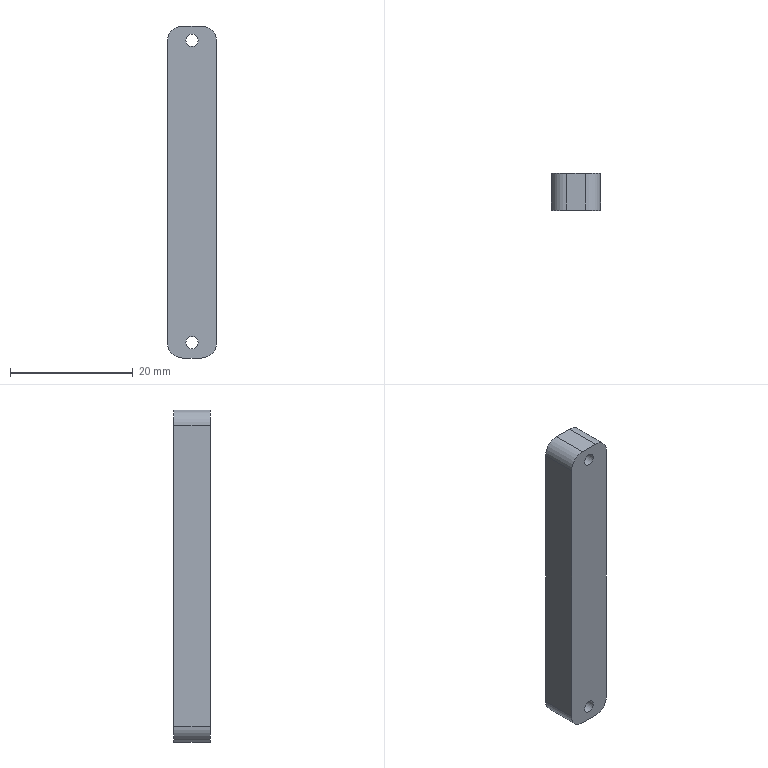Component | NX | ROBOT_ARM_LONG_ARM | 1 solid | 12 faces | box 8 x 6 x 54 mm | volume 2522 mm3 | plane 6 | cylinder 6 | commonest cylinder face diameters 5 x4 2 x2
STEP:
#1=CARTESIAN_POINT('',(0.,0.,0.));
#2=DIRECTION('',(0.,0.,1.));
#3=DIRECTION('',(1.,0.,0.));
#4=AXIS2_PLACEMENT_3D('',#1,#2,#3);
#5=CARTESIAN_POINT('',(7.471,23.498,87.5));
#6=VERTEX_POINT('',#5);
#7=CARTESIAN_POINT('',(7.471,23.498,38.5));
#8=VERTEX_POINT('',#7);
#9=CARTESIAN_POINT('',(7.471,23.498,87.5));
#10=DIRECTION('',(0.,0.,-1.));
#11=VECTOR('',#10,1.);
#12=LINE('',#9,#11);
#13=CARTESIAN_POINT('',(7.471,17.498,87.5));
#14=DIRECTION('',(1.,0.,0.));
#15=DIRECTION('',(-0.,0.,1.));
#16=AXIS2_PLACEMENT_3D('',#13,#14,#15);
#17=PLANE('',#16);
#18=CARTESIAN_POINT('',(0.,-6.));
#19=DIRECTION('',(-1.,0.));
#20=VECTOR('',#19,1.);
#21=LINE('',#18,#20);
#22=(GEOMETRIC_REPRESENTATION_CONTEXT(2)PARAMETRIC_REPRESENTATION_CONTEXT()REPRESENTATION_CONTEXT('',''));
#23=DEFINITIONAL_REPRESENTATION('',(#21),#22);
#24=PCURVE('',#17,#23);
#25=CARTESIAN_POINT('',(9.971,23.498,38.5));
#26=DIRECTION('',(0.,-1.,0.));
#27=DIRECTION('',(1.,0.,0.));
#28=AXIS2_PLACEMENT_3D('',#25,#26,#27);
#29=PLANE('',#28);
#30=CARTESIAN_POINT('',(-2.5,49.));
#31=DIRECTION('',(0.,-1.));
#32=VECTOR('',#31,1.);
#33=LINE('',#30,#32);
#34=(GEOMETRIC_REPRESENTATION_CONTEXT(2)PARAMETRIC_REPRESENTATION_CONTEXT()REPRESENTATION_CONTEXT('',''));
#35=DEFINITIONAL_REPRESENTATION('',(#33),#34);
#36=PCURVE('',#29,#35);
#37=SURFACE_CURVE('',#12,(#24,#36),.PCURVE_S1.);
#38=EDGE_CURVE('',#6,#8,#37,.T.);
#39=ORIENTED_EDGE('',*,*,#38,.T.);
#40=CARTESIAN_POINT('',(7.471,17.498,38.5));
#41=VERTEX_POINT('',#40);
#42=CARTESIAN_POINT('',(7.471,17.498,38.5));
#43=DIRECTION('',(0.,1.,0.));
#44=VECTOR('',#43,1.);
#45=LINE('',#42,#44);
#46=CARTESIAN_POINT('',(-49.,0.));
#47=DIRECTION('',(0.,-1.));
#48=VECTOR('',#47,1.);
#49=LINE('',#46,#48);
#50=(GEOMETRIC_REPRESENTATION_CONTEXT(2)PARAMETRIC_REPRESENTATION_CONTEXT()REPRESENTATION_CONTEXT('',''));
#51=DEFINITIONAL_REPRESENTATION('',(#49),#50);
#52=PCURVE('',#17,#51);
#53=CARTESIAN_POINT('',(9.971,17.498,38.5));
#54=DIRECTION('',(0.,1.,0.));
#55=DIRECTION('',(-1.,0.,0.));
#56=AXIS2_PLACEMENT_3D('',#53,#54,#55);
#57=CYLINDRICAL_SURFACE('',#56,2.5);
#58=CARTESIAN_POINT('',(6.283,0.));
#59=DIRECTION('',(0.,1.));
#60=VECTOR('',#59,1.);
#61=LINE('',#58,#60);
#62=(GEOMETRIC_REPRESENTATION_CONTEXT(2)PARAMETRIC_REPRESENTATION_CONTEXT()REPRESENTATION_CONTEXT('',''));
#63=DEFINITIONAL_REPRESENTATION('',(#61),#62);
#64=PCURVE('',#57,#63);
#65=SURFACE_CURVE('',#45,(#52,#64),.PCURVE_S1.);
#66=EDGE_CURVE('',#41,#8,#65,.T.);
#67=ORIENTED_EDGE('',*,*,#66,.F.);
#68=CARTESIAN_POINT('',(7.471,17.498,87.5));
#69=VERTEX_POINT('',#68);
#70=CARTESIAN_POINT('',(7.471,17.498,87.5));
#71=DIRECTION('',(0.,0.,-1.));
#72=VECTOR('',#71,1.);
#73=LINE('',#70,#72);
#74=CARTESIAN_POINT('',(0.,0.));
#75=DIRECTION('',(-1.,0.));
#76=VECTOR('',#75,1.);
#77=LINE('',#74,#76);
#78=(GEOMETRIC_REPRESENTATION_CONTEXT(2)PARAMETRIC_REPRESENTATION_CONTEXT()REPRESENTATION_CONTEXT('',''));
#79=DEFINITIONAL_REPRESENTATION('',(#77),#78);
#80=PCURVE('',#17,#79);
#81=CARTESIAN_POINT('',(9.971,17.498,38.5));
#82=DIRECTION('',(0.,-1.,0.));
#83=DIRECTION('',(1.,0.,0.));
#84=AXIS2_PLACEMENT_3D('',#81,#82,#83);
#85=PLANE('',#84);
#86=CARTESIAN_POINT('',(-2.5,49.));
#87=DIRECTION('',(0.,-1.));
#88=VECTOR('',#87,1.);
#89=LINE('',#86,#88);
#90=(GEOMETRIC_REPRESENTATION_CONTEXT(2)PARAMETRIC_REPRESENTATION_CONTEXT()REPRESENTATION_CONTEXT('',''));
#91=DEFINITIONAL_REPRESENTATION('',(#89),#90);
#92=PCURVE('',#85,#91);
#93=SURFACE_CURVE('',#73,(#80,#92),.PCURVE_S1.);
#94=EDGE_CURVE('',#69,#41,#93,.T.);
#95=ORIENTED_EDGE('',*,*,#94,.F.);
#96=CARTESIAN_POINT('',(7.471,17.498,87.5));
#97=DIRECTION('',(0.,1.,0.));
#98=VECTOR('',#97,1.);
#99=LINE('',#96,#98);
#100=CARTESIAN_POINT('',(0.,0.));
#101=DIRECTION('',(0.,-1.));
#102=VECTOR('',#101,1.);
#103=LINE('',#100,#102);
#104=(GEOMETRIC_REPRESENTATION_CONTEXT(2)PARAMETRIC_REPRESENTATION_CONTEXT()REPRESENTATION_CONTEXT('',''));
#105=DEFINITIONAL_REPRESENTATION('',(#103),#104);
#106=PCURVE('',#17,#105);
#107=CARTESIAN_POINT('',(9.971,17.498,87.5));
#108=DIRECTION('',(0.,1.,0.));
#109=DIRECTION('',(-1.,0.,0.));
#110=AXIS2_PLACEMENT_3D('',#107,#108,#109);
#111=CYLINDRICAL_SURFACE('',#110,2.5);
#112=CARTESIAN_POINT('',(0.,0.));
#113=DIRECTION('',(0.,1.));
#114=VECTOR('',#113,1.);
#115=LINE('',#112,#114);
#116=(GEOMETRIC_REPRESENTATION_CONTEXT(2)PARAMETRIC_REPRESENTATION_CONTEXT()REPRESENTATION_CONTEXT('',''));
#117=DEFINITIONAL_REPRESENTATION('',(#115),#116);
#118=PCURVE('',#111,#117);
#119=SURFACE_CURVE('',#99,(#106,#118),.PCURVE_S1.);
#120=EDGE_CURVE('',#69,#6,#119,.T.);
#121=ORIENTED_EDGE('',*,*,#120,.T.);
#122=EDGE_LOOP('',(#39,#67,#95,#121));
#123=FACE_BOUND('',#122,.T.);
#124=ADVANCED_FACE('',(#123),#17,.F.);
#125=CARTESIAN_POINT('',(9.971,23.498,36.));
#126=VERTEX_POINT('',#125);
#127=CARTESIAN_POINT('',(9.971,23.498,38.5));
#128=DIRECTION('',(0.,-1.,0.));
#129=DIRECTION('',(1.,0.,0.));
#130=AXIS2_PLACEMENT_3D('',#127,#128,#129);
#131=CIRCLE('',#130,2.5);
#132=CARTESIAN_POINT('',(9.425,6.));
#133=DIRECTION('',(-1.,0.));
#134=VECTOR('',#133,1.);
#135=LINE('',#132,#134);
#136=(GEOMETRIC_REPRESENTATION_CONTEXT(2)PARAMETRIC_REPRESENTATION_CONTEXT()REPRESENTATION_CONTEXT('',''));
#137=DEFINITIONAL_REPRESENTATION('',(#135),#136);
#138=PCURVE('',#57,#137);
#139=CARTESIAN_POINT('',(0.,0.));
#140=DIRECTION('',(1.,0.));
#141=AXIS2_PLACEMENT_2D('',#139,#140);
#142=CIRCLE('',#141,2.5);
#143=(GEOMETRIC_REPRESENTATION_CONTEXT(2)PARAMETRIC_REPRESENTATION_CONTEXT()REPRESENTATION_CONTEXT('',''));
#144=DEFINITIONAL_REPRESENTATION('',(#142),#143);
#145=PCURVE('',#29,#144);
#146=SURFACE_CURVE('',#131,(#138,#145),.PCURVE_S1.);
#147=EDGE_CURVE('',#8,#126,#146,.T.);
#148=ORIENTED_EDGE('',*,*,#147,.T.);
#149=CARTESIAN_POINT('',(9.971,17.498,36.));
#150=VERTEX_POINT('',#149);
#151=CARTESIAN_POINT('',(9.971,17.498,36.));
#152=DIRECTION('',(0.,1.,0.));
#153=VECTOR('',#152,1.);
#154=LINE('',#151,#153);
#155=CARTESIAN_POINT('',(4.712,0.));
#156=DIRECTION('',(0.,1.));
#157=VECTOR('',#156,1.);
#158=LINE('',#155,#157);
#159=(GEOMETRIC_REPRESENTATION_CONTEXT(2)PARAMETRIC_REPRESENTATION_CONTEXT()REPRESENTATION_CONTEXT('',''));
#160=DEFINITIONAL_REPRESENTATION('',(#158),#159);
#161=PCURVE('',#57,#160);
#162=CARTESIAN_POINT('',(9.971,17.498,36.));
#163=DIRECTION('',(0.,0.,1.));
#164=DIRECTION('',(0.,-1.,0.));
#165=AXIS2_PLACEMENT_3D('',#162,#163,#164);
#166=PLANE('',#165);
#167=CARTESIAN_POINT('',(0.,0.));
#168=DIRECTION('',(-1.,0.));
#169=VECTOR('',#168,1.);
#170=LINE('',#167,#169);
#171=(GEOMETRIC_REPRESENTATION_CONTEXT(2)PARAMETRIC_REPRESENTATION_CONTEXT()REPRESENTATION_CONTEXT('',''));
#172=DEFINITIONAL_REPRESENTATION('',(#170),#171);
#173=PCURVE('',#166,#172);
#174=SURFACE_CURVE('',#154,(#161,#173),.PCURVE_S1.);
#175=EDGE_CURVE('',#150,#126,#174,.T.);
#176=ORIENTED_EDGE('',*,*,#175,.F.);
#177=CARTESIAN_POINT('',(9.971,17.498,38.5));
#178=DIRECTION('',(0.,-1.,0.));
#179=DIRECTION('',(1.,0.,0.));
#180=AXIS2_PLACEMENT_3D('',#177,#178,#179);
#181=CIRCLE('',#180,2.5);
#182=CARTESIAN_POINT('',(9.425,0.));
#183=DIRECTION('',(-1.,0.));
#184=VECTOR('',#183,1.);
#185=LINE('',#182,#184);
#186=(GEOMETRIC_REPRESENTATION_CONTEXT(2)PARAMETRIC_REPRESENTATION_CONTEXT()REPRESENTATION_CONTEXT('',''));
#187=DEFINITIONAL_REPRESENTATION('',(#185),#186);
#188=PCURVE('',#57,#187);
#189=CARTESIAN_POINT('',(0.,0.));
#190=DIRECTION('',(1.,0.));
#191=AXIS2_PLACEMENT_2D('',#189,#190);
#192=CIRCLE('',#191,2.5);
#193=(GEOMETRIC_REPRESENTATION_CONTEXT(2)PARAMETRIC_REPRESENTATION_CONTEXT()REPRESENTATION_CONTEXT('',''));
#194=DEFINITIONAL_REPRESENTATION('',(#192),#193);
#195=PCURVE('',#85,#194);
#196=SURFACE_CURVE('',#181,(#188,#195),.PCURVE_S1.);
#197=EDGE_CURVE('',#41,#150,#196,.T.);
#198=ORIENTED_EDGE('',*,*,#197,.F.);
#199=ORIENTED_EDGE('',*,*,#66,.T.);
#200=EDGE_LOOP('',(#148,#176,#198,#199));
#201=FACE_BOUND('',#200,.T.);
#202=ADVANCED_FACE('',(#201),#57,.T.);
#203=CARTESIAN_POINT('',(12.971,23.498,36.));
#204=VERTEX_POINT('',#203);
#205=CARTESIAN_POINT('',(9.971,23.498,36.));
#206=DIRECTION('',(1.,0.,0.));
#207=VECTOR('',#206,1.);
#208=LINE('',#205,#207);
#209=CARTESIAN_POINT('',(-6.,0.));
#210=DIRECTION('',(0.,1.));
#211=VECTOR('',#210,1.);
#212=LINE('',#209,#211);
#213=(GEOMETRIC_REPRESENTATION_CONTEXT(2)PARAMETRIC_REPRESENTATION_CONTEXT()REPRESENTATION_CONTEXT('',''));
#214=DEFINITIONAL_REPRESENTATION('',(#212),#213);
#215=PCURVE('',#166,#214);
#216=CARTESIAN_POINT('',(0.,-2.5));
#217=DIRECTION('',(1.,0.));
#218=VECTOR('',#217,1.);
#219=LINE('',#216,#218);
#220=(GEOMETRIC_REPRESENTATION_CONTEXT(2)PARAMETRIC_REPRESENTATION_CONTEXT()REPRESENTATION_CONTEXT('',''));
#221=DEFINITIONAL_REPRESENTATION('',(#219),#220);
#222=PCURVE('',#29,#221);
#223=SURFACE_CURVE('',#208,(#215,#222),.PCURVE_S1.);
#224=EDGE_CURVE('',#126,#204,#223,.T.);
#225=ORIENTED_EDGE('',*,*,#224,.T.);
#226=CARTESIAN_POINT('',(12.971,17.498,36.));
#227=VERTEX_POINT('',#226);
#228=CARTESIAN_POINT('',(12.971,17.498,36.));
#229=DIRECTION('',(0.,1.,0.));
#230=VECTOR('',#229,1.);
#231=LINE('',#228,#230);
#232=CARTESIAN_POINT('',(0.,3.));
#233=DIRECTION('',(-1.,0.));
#234=VECTOR('',#233,1.);
#235=LINE('',#232,#234);
#236=(GEOMETRIC_REPRESENTATION_CONTEXT(2)PARAMETRIC_REPRESENTATION_CONTEXT()REPRESENTATION_CONTEXT('',''));
#237=DEFINITIONAL_REPRESENTATION('',(#235),#236);
#238=PCURVE('',#166,#237);
#239=CARTESIAN_POINT('',(12.971,17.498,38.5));
#240=DIRECTION('',(0.,1.,0.));
#241=DIRECTION('',(-1.,0.,0.));
#242=AXIS2_PLACEMENT_3D('',#239,#240,#241);
#243=CYLINDRICAL_SURFACE('',#242,2.5);
#244=CARTESIAN_POINT('',(4.712,0.));
#245=DIRECTION('',(0.,1.));
#246=VECTOR('',#245,1.);
#247=LINE('',#244,#246);
#248=(GEOMETRIC_REPRESENTATION_CONTEXT(2)PARAMETRIC_REPRESENTATION_CONTEXT()REPRESENTATION_CONTEXT('',''));
#249=DEFINITIONAL_REPRESENTATION('',(#247),#248);
#250=PCURVE('',#243,#249);
#251=SURFACE_CURVE('',#231,(#238,#250),.PCURVE_S1.);
#252=EDGE_CURVE('',#227,#204,#251,.T.);
#253=ORIENTED_EDGE('',*,*,#252,.F.);
#254=CARTESIAN_POINT('',(9.971,17.498,36.));
#255=DIRECTION('',(1.,0.,0.));
#256=VECTOR('',#255,1.);
#257=LINE('',#254,#256);
#258=CARTESIAN_POINT('',(0.,0.));
#259=DIRECTION('',(0.,1.));
#260=VECTOR('',#259,1.);
#261=LINE('',#258,#260);
#262=(GEOMETRIC_REPRESENTATION_CONTEXT(2)PARAMETRIC_REPRESENTATION_CONTEXT()REPRESENTATION_CONTEXT('',''));
#263=DEFINITIONAL_REPRESENTATION('',(#261),#262);
#264=PCURVE('',#166,#263);
#265=CARTESIAN_POINT('',(0.,-2.5));
#266=DIRECTION('',(1.,0.));
#267=VECTOR('',#266,1.);
#268=LINE('',#265,#267);
#269=(GEOMETRIC_REPRESENTATION_CONTEXT(2)PARAMETRIC_REPRESENTATION_CONTEXT()REPRESENTATION_CONTEXT('',''));
#270=DEFINITIONAL_REPRESENTATION('',(#268),#269);
#271=PCURVE('',#85,#270);
#272=SURFACE_CURVE('',#257,(#264,#271),.PCURVE_S1.);
#273=EDGE_CURVE('',#150,#227,#272,.T.);
#274=ORIENTED_EDGE('',*,*,#273,.F.);
#275=ORIENTED_EDGE('',*,*,#175,.T.);
#276=EDGE_LOOP('',(#225,#253,#274,#275));
#277=FACE_BOUND('',#276,.T.);
#278=ADVANCED_FACE('',(#277),#166,.F.);
#279=CARTESIAN_POINT('',(15.471,23.498,38.5));
#280=VERTEX_POINT('',#279);
#281=CARTESIAN_POINT('',(12.971,23.498,38.5));
#282=DIRECTION('',(0.,-1.,0.));
#283=DIRECTION('',(1.,0.,0.));
#284=AXIS2_PLACEMENT_3D('',#281,#282,#283);
#285=CIRCLE('',#284,2.5);
#286=CARTESIAN_POINT('',(9.425,6.));
#287=DIRECTION('',(-1.,0.));
#288=VECTOR('',#287,1.);
#289=LINE('',#286,#288);
#290=(GEOMETRIC_REPRESENTATION_CONTEXT(2)PARAMETRIC_REPRESENTATION_CONTEXT()REPRESENTATION_CONTEXT('',''));
#291=DEFINITIONAL_REPRESENTATION('',(#289),#290);
#292=PCURVE('',#243,#291);
#293=CARTESIAN_POINT('',(3.,0.));
#294=DIRECTION('',(1.,0.));
#295=AXIS2_PLACEMENT_2D('',#293,#294);
#296=CIRCLE('',#295,2.5);
#297=(GEOMETRIC_REPRESENTATION_CONTEXT(2)PARAMETRIC_REPRESENTATION_CONTEXT()REPRESENTATION_CONTEXT('',''));
#298=DEFINITIONAL_REPRESENTATION('',(#296),#297);
#299=PCURVE('',#29,#298);
#300=SURFACE_CURVE('',#285,(#292,#299),.PCURVE_S1.);
#301=EDGE_CURVE('',#204,#280,#300,.T.);
#302=ORIENTED_EDGE('',*,*,#301,.T.);
#303=CARTESIAN_POINT('',(15.471,17.498,38.5));
#304=VERTEX_POINT('',#303);
#305=CARTESIAN_POINT('',(15.471,17.498,38.5));
#306=DIRECTION('',(0.,1.,0.));
#307=VECTOR('',#306,1.);
#308=LINE('',#305,#307);
#309=CARTESIAN_POINT('',(3.142,0.));
#310=DIRECTION('',(0.,1.));
#311=VECTOR('',#310,1.);
#312=LINE('',#309,#311);
#313=(GEOMETRIC_REPRESENTATION_CONTEXT(2)PARAMETRIC_REPRESENTATION_CONTEXT()REPRESENTATION_CONTEXT('',''));
#314=DEFINITIONAL_REPRESENTATION('',(#312),#313);
#315=PCURVE('',#243,#314);
#316=CARTESIAN_POINT('',(15.471,17.498,38.5));
#317=DIRECTION('',(-1.,0.,-0.));
#318=DIRECTION('',(0.,0.,-1.));
#319=AXIS2_PLACEMENT_3D('',#316,#317,#318);
#320=PLANE('',#319);
#321=CARTESIAN_POINT('',(0.,0.));
#322=DIRECTION('',(0.,-1.));
#323=VECTOR('',#322,1.);
#324=LINE('',#321,#323);
#325=(GEOMETRIC_REPRESENTATION_CONTEXT(2)PARAMETRIC_REPRESENTATION_CONTEXT()REPRESENTATION_CONTEXT('',''));
#326=DEFINITIONAL_REPRESENTATION('',(#324),#325);
#327=PCURVE('',#320,#326);
#328=SURFACE_CURVE('',#308,(#315,#327),.PCURVE_S1.);
#329=EDGE_CURVE('',#304,#280,#328,.T.);
#330=ORIENTED_EDGE('',*,*,#329,.F.);
#331=CARTESIAN_POINT('',(12.971,17.498,38.5));
#332=DIRECTION('',(0.,-1.,0.));
#333=DIRECTION('',(1.,0.,0.));
#334=AXIS2_PLACEMENT_3D('',#331,#332,#333);
#335=CIRCLE('',#334,2.5);
#336=CARTESIAN_POINT('',(9.425,0.));
#337=DIRECTION('',(-1.,0.));
#338=VECTOR('',#337,1.);
#339=LINE('',#336,#338);
#340=(GEOMETRIC_REPRESENTATION_CONTEXT(2)PARAMETRIC_REPRESENTATION_CONTEXT()REPRESENTATION_CONTEXT('',''));
#341=DEFINITIONAL_REPRESENTATION('',(#339),#340);
#342=PCURVE('',#243,#341);
#343=CARTESIAN_POINT('',(3.,0.));
#344=DIRECTION('',(1.,0.));
#345=AXIS2_PLACEMENT_2D('',#343,#344);
#346=CIRCLE('',#345,2.5);
#347=(GEOMETRIC_REPRESENTATION_CONTEXT(2)PARAMETRIC_REPRESENTATION_CONTEXT()REPRESENTATION_CONTEXT('',''));
#348=DEFINITIONAL_REPRESENTATION('',(#346),#347);
#349=PCURVE('',#85,#348);
#350=SURFACE_CURVE('',#335,(#342,#349),.PCURVE_S1.);
#351=EDGE_CURVE('',#227,#304,#350,.T.);
#352=ORIENTED_EDGE('',*,*,#351,.F.);
#353=ORIENTED_EDGE('',*,*,#252,.T.);
#354=EDGE_LOOP('',(#302,#330,#352,#353));
#355=FACE_BOUND('',#354,.T.);
#356=ADVANCED_FACE('',(#355),#243,.T.);
#357=CARTESIAN_POINT('',(15.471,23.498,87.5));
#358=VERTEX_POINT('',#357);
#359=CARTESIAN_POINT('',(15.471,23.498,38.5));
#360=DIRECTION('',(-0.,0.,1.));
#361=VECTOR('',#360,1.);
#362=LINE('',#359,#361);
#363=CARTESIAN_POINT('',(0.,-6.));
#364=DIRECTION('',(-1.,0.));
#365=VECTOR('',#364,1.);
#366=LINE('',#363,#365);
#367=(GEOMETRIC_REPRESENTATION_CONTEXT(2)PARAMETRIC_REPRESENTATION_CONTEXT()REPRESENTATION_CONTEXT('',''));
#368=DEFINITIONAL_REPRESENTATION('',(#366),#367);
#369=PCURVE('',#320,#368);
#370=CARTESIAN_POINT('',(5.5,0.));
#371=DIRECTION('',(-0.,1.));
#372=VECTOR('',#371,1.);
#373=LINE('',#370,#372);
#374=(GEOMETRIC_REPRESENTATION_CONTEXT(2)PARAMETRIC_REPRESENTATION_CONTEXT()REPRESENTATION_CONTEXT('',''));
#375=DEFINITIONAL_REPRESENTATION('',(#373),#374);
#376=PCURVE('',#29,#375);
#377=SURFACE_CURVE('',#362,(#369,#376),.PCURVE_S1.);
#378=EDGE_CURVE('',#280,#358,#377,.T.);
#379=ORIENTED_EDGE('',*,*,#378,.T.);
#380=CARTESIAN_POINT('',(15.471,17.498,87.5));
#381=VERTEX_POINT('',#380);
#382=CARTESIAN_POINT('',(15.471,17.498,87.5));
#383=DIRECTION('',(0.,1.,0.));
#384=VECTOR('',#383,1.);
#385=LINE('',#382,#384);
#386=CARTESIAN_POINT('',(-49.,0.));
#387=DIRECTION('',(0.,-1.));
#388=VECTOR('',#387,1.);
#389=LINE('',#386,#388);
#390=(GEOMETRIC_REPRESENTATION_CONTEXT(2)PARAMETRIC_REPRESENTATION_CONTEXT()REPRESENTATION_CONTEXT('',''));
#391=DEFINITIONAL_REPRESENTATION('',(#389),#390);
#392=PCURVE('',#320,#391);
#393=CARTESIAN_POINT('',(12.971,17.498,87.5));
#394=DIRECTION('',(0.,1.,0.));
#395=DIRECTION('',(-1.,0.,0.));
#396=AXIS2_PLACEMENT_3D('',#393,#394,#395);
#397=CYLINDRICAL_SURFACE('',#396,2.5);
#398=CARTESIAN_POINT('',(3.142,0.));
#399=DIRECTION('',(0.,1.));
#400=VECTOR('',#399,1.);
#401=LINE('',#398,#400);
#402=(GEOMETRIC_REPRESENTATION_CONTEXT(2)PARAMETRIC_REPRESENTATION_CONTEXT()REPRESENTATION_CONTEXT('',''));
#403=DEFINITIONAL_REPRESENTATION('',(#401),#402);
#404=PCURVE('',#397,#403);
#405=SURFACE_CURVE('',#385,(#392,#404),.PCURVE_S1.);
#406=EDGE_CURVE('',#381,#358,#405,.T.);
#407=ORIENTED_EDGE('',*,*,#406,.F.);
#408=CARTESIAN_POINT('',(15.471,17.498,38.5));
#409=DIRECTION('',(-0.,0.,1.));
#410=VECTOR('',#409,1.);
#411=LINE('',#408,#410);
#412=CARTESIAN_POINT('',(0.,0.));
#413=DIRECTION('',(-1.,0.));
#414=VECTOR('',#413,1.);
#415=LINE('',#412,#414);
#416=(GEOMETRIC_REPRESENTATION_CONTEXT(2)PARAMETRIC_REPRESENTATION_CONTEXT()REPRESENTATION_CONTEXT('',''));
#417=DEFINITIONAL_REPRESENTATION('',(#415),#416);
#418=PCURVE('',#320,#417);
#419=CARTESIAN_POINT('',(5.5,0.));
#420=DIRECTION('',(-0.,1.));
#421=VECTOR('',#420,1.);
#422=LINE('',#419,#421);
#423=(GEOMETRIC_REPRESENTATION_CONTEXT(2)PARAMETRIC_REPRESENTATION_CONTEXT()REPRESENTATION_CONTEXT('',''));
#424=DEFINITIONAL_REPRESENTATION('',(#422),#423);
#425=PCURVE('',#85,#424);
#426=SURFACE_CURVE('',#411,(#418,#425),.PCURVE_S1.);
#427=EDGE_CURVE('',#304,#381,#426,.T.);
#428=ORIENTED_EDGE('',*,*,#427,.F.);
#429=ORIENTED_EDGE('',*,*,#329,.T.);
#430=EDGE_LOOP('',(#379,#407,#428,#429));
#431=FACE_BOUND('',#430,.T.);
#432=ADVANCED_FACE('',(#431),#320,.F.);
#433=CARTESIAN_POINT('',(12.971,23.498,90.));
#434=VERTEX_POINT('',#433);
#435=CARTESIAN_POINT('',(12.971,23.498,87.5));
#436=DIRECTION('',(0.,-1.,0.));
#437=DIRECTION('',(1.,0.,0.));
#438=AXIS2_PLACEMENT_3D('',#435,#436,#437);
#439=CIRCLE('',#438,2.5);
#440=CARTESIAN_POINT('',(3.142,6.));
#441=DIRECTION('',(-1.,0.));
#442=VECTOR('',#441,1.);
#443=LINE('',#440,#442);
#444=(GEOMETRIC_REPRESENTATION_CONTEXT(2)PARAMETRIC_REPRESENTATION_CONTEXT()REPRESENTATION_CONTEXT('',''));
#445=DEFINITIONAL_REPRESENTATION('',(#443),#444);
#446=PCURVE('',#397,#445);
#447=CARTESIAN_POINT('',(3.,49.));
#448=DIRECTION('',(1.,0.));
#449=AXIS2_PLACEMENT_2D('',#447,#448);
#450=CIRCLE('',#449,2.5);
#451=(GEOMETRIC_REPRESENTATION_CONTEXT(2)PARAMETRIC_REPRESENTATION_CONTEXT()REPRESENTATION_CONTEXT('',''));
#452=DEFINITIONAL_REPRESENTATION('',(#450),#451);
#453=PCURVE('',#29,#452);
#454=SURFACE_CURVE('',#439,(#446,#453),.PCURVE_S1.);
#455=EDGE_CURVE('',#358,#434,#454,.T.);
#456=ORIENTED_EDGE('',*,*,#455,.T.);
#457=CARTESIAN_POINT('',(12.971,17.498,90.));
#458=VERTEX_POINT('',#457);
#459=CARTESIAN_POINT('',(12.971,17.498,90.));
#460=DIRECTION('',(0.,1.,0.));
#461=VECTOR('',#460,1.);
#462=LINE('',#459,#461);
#463=CARTESIAN_POINT('',(1.571,0.));
#464=DIRECTION('',(0.,1.));
#465=VECTOR('',#464,1.);
#466=LINE('',#463,#465);
#467=(GEOMETRIC_REPRESENTATION_CONTEXT(2)PARAMETRIC_REPRESENTATION_CONTEXT()REPRESENTATION_CONTEXT('',''));
#468=DEFINITIONAL_REPRESENTATION('',(#466),#467);
#469=PCURVE('',#397,#468);
#470=CARTESIAN_POINT('',(12.971,17.498,90.));
#471=DIRECTION('',(0.,0.,-1.));
#472=DIRECTION('',(0.,1.,0.));
#473=AXIS2_PLACEMENT_3D('',#470,#471,#472);
#474=PLANE('',#473);
#475=CARTESIAN_POINT('',(0.,0.));
#476=DIRECTION('',(1.,0.));
#477=VECTOR('',#476,1.);
#478=LINE('',#475,#477);
#479=(GEOMETRIC_REPRESENTATION_CONTEXT(2)PARAMETRIC_REPRESENTATION_CONTEXT()REPRESENTATION_CONTEXT('',''));
#480=DEFINITIONAL_REPRESENTATION('',(#478),#479);
#481=PCURVE('',#474,#480);
#482=SURFACE_CURVE('',#462,(#469,#481),.PCURVE_S1.);
#483=EDGE_CURVE('',#458,#434,#482,.T.);
#484=ORIENTED_EDGE('',*,*,#483,.F.);
#485=CARTESIAN_POINT('',(12.971,17.498,87.5));
#486=DIRECTION('',(0.,-1.,0.));
#487=DIRECTION('',(1.,0.,0.));
#488=AXIS2_PLACEMENT_3D('',#485,#486,#487);
#489=CIRCLE('',#488,2.5);
#490=CARTESIAN_POINT('',(3.142,0.));
#491=DIRECTION('',(-1.,0.));
#492=VECTOR('',#491,1.);
#493=LINE('',#490,#492);
#494=(GEOMETRIC_REPRESENTATION_CONTEXT(2)PARAMETRIC_REPRESENTATION_CONTEXT()REPRESENTATION_CONTEXT('',''));
#495=DEFINITIONAL_REPRESENTATION('',(#493),#494);
#496=PCURVE('',#397,#495);
#497=CARTESIAN_POINT('',(3.,49.));
#498=DIRECTION('',(1.,0.));
#499=AXIS2_PLACEMENT_2D('',#497,#498);
#500=CIRCLE('',#499,2.5);
#501=(GEOMETRIC_REPRESENTATION_CONTEXT(2)PARAMETRIC_REPRESENTATION_CONTEXT()REPRESENTATION_CONTEXT('',''));
#502=DEFINITIONAL_REPRESENTATION('',(#500),#501);
#503=PCURVE('',#85,#502);
#504=SURFACE_CURVE('',#489,(#496,#503),.PCURVE_S1.);
#505=EDGE_CURVE('',#381,#458,#504,.T.);
#506=ORIENTED_EDGE('',*,*,#505,.F.);
#507=ORIENTED_EDGE('',*,*,#406,.T.);
#508=EDGE_LOOP('',(#456,#484,#506,#507));
#509=FACE_BOUND('',#508,.T.);
#510=ADVANCED_FACE('',(#509),#397,.T.);
#511=CARTESIAN_POINT('',(9.971,23.498,90.));
#512=VERTEX_POINT('',#511);
#513=CARTESIAN_POINT('',(12.971,23.498,90.));
#514=DIRECTION('',(-1.,0.,0.));
#515=VECTOR('',#514,1.);
#516=LINE('',#513,#515);
#517=CARTESIAN_POINT('',(6.,0.));
#518=DIRECTION('',(0.,-1.));
#519=VECTOR('',#518,1.);
#520=LINE('',#517,#519);
#521=(GEOMETRIC_REPRESENTATION_CONTEXT(2)PARAMETRIC_REPRESENTATION_CONTEXT()REPRESENTATION_CONTEXT('',''));
#522=DEFINITIONAL_REPRESENTATION('',(#520),#521);
#523=PCURVE('',#474,#522);
#524=CARTESIAN_POINT('',(3.,51.5));
#525=DIRECTION('',(-1.,0.));
#526=VECTOR('',#525,1.);
#527=LINE('',#524,#526);
#528=(GEOMETRIC_REPRESENTATION_CONTEXT(2)PARAMETRIC_REPRESENTATION_CONTEXT()REPRESENTATION_CONTEXT('',''));
#529=DEFINITIONAL_REPRESENTATION('',(#527),#528);
#530=PCURVE('',#29,#529);
#531=SURFACE_CURVE('',#516,(#523,#530),.PCURVE_S1.);
#532=EDGE_CURVE('',#434,#512,#531,.T.);
#533=ORIENTED_EDGE('',*,*,#532,.T.);
#534=CARTESIAN_POINT('',(9.971,17.498,90.));
#535=VERTEX_POINT('',#534);
#536=CARTESIAN_POINT('',(9.971,17.498,90.));
#537=DIRECTION('',(0.,1.,0.));
#538=VECTOR('',#537,1.);
#539=LINE('',#536,#538);
#540=CARTESIAN_POINT('',(0.,-3.));
#541=DIRECTION('',(1.,0.));
#542=VECTOR('',#541,1.);
#543=LINE('',#540,#542);
#544=(GEOMETRIC_REPRESENTATION_CONTEXT(2)PARAMETRIC_REPRESENTATION_CONTEXT()REPRESENTATION_CONTEXT('',''));
#545=DEFINITIONAL_REPRESENTATION('',(#543),#544);
#546=PCURVE('',#474,#545);
#547=CARTESIAN_POINT('',(1.571,0.));
#548=DIRECTION('',(0.,1.));
#549=VECTOR('',#548,1.);
#550=LINE('',#547,#549);
#551=(GEOMETRIC_REPRESENTATION_CONTEXT(2)PARAMETRIC_REPRESENTATION_CONTEXT()REPRESENTATION_CONTEXT('',''));
#552=DEFINITIONAL_REPRESENTATION('',(#550),#551);
#553=PCURVE('',#111,#552);
#554=SURFACE_CURVE('',#539,(#546,#553),.PCURVE_S1.);
#555=EDGE_CURVE('',#535,#512,#554,.T.);
#556=ORIENTED_EDGE('',*,*,#555,.F.);
#557=CARTESIAN_POINT('',(12.971,17.498,90.));
#558=DIRECTION('',(-1.,0.,0.));
#559=VECTOR('',#558,1.);
#560=LINE('',#557,#559);
#561=CARTESIAN_POINT('',(0.,0.));
#562=DIRECTION('',(0.,-1.));
#563=VECTOR('',#562,1.);
#564=LINE('',#561,#563);
#565=(GEOMETRIC_REPRESENTATION_CONTEXT(2)PARAMETRIC_REPRESENTATION_CONTEXT()REPRESENTATION_CONTEXT('',''));
#566=DEFINITIONAL_REPRESENTATION('',(#564),#565);
#567=PCURVE('',#474,#566);
#568=CARTESIAN_POINT('',(3.,51.5));
#569=DIRECTION('',(-1.,0.));
#570=VECTOR('',#569,1.);
#571=LINE('',#568,#570);
#572=(GEOMETRIC_REPRESENTATION_CONTEXT(2)PARAMETRIC_REPRESENTATION_CONTEXT()REPRESENTATION_CONTEXT('',''));
#573=DEFINITIONAL_REPRESENTATION('',(#571),#572);
#574=PCURVE('',#85,#573);
#575=SURFACE_CURVE('',#560,(#567,#574),.PCURVE_S1.);
#576=EDGE_CURVE('',#458,#535,#575,.T.);
#577=ORIENTED_EDGE('',*,*,#576,.F.);
#578=ORIENTED_EDGE('',*,*,#483,.T.);
#579=EDGE_LOOP('',(#533,#556,#577,#578));
#580=FACE_BOUND('',#579,.T.);
#581=ADVANCED_FACE('',(#580),#474,.F.);
#582=CARTESIAN_POINT('',(12.471,17.498,38.5));
#583=VERTEX_POINT('',#582);
#584=CARTESIAN_POINT('',(11.471,17.498,38.5));
#585=DIRECTION('',(0.,-1.,0.));
#586=DIRECTION('',(1.,0.,0.));
#587=AXIS2_PLACEMENT_3D('',#584,#585,#586);
#588=CIRCLE('',#587,1.);
#589=CARTESIAN_POINT('',(11.471,17.498,38.5));
#590=DIRECTION('',(0.,1.,0.));
#591=DIRECTION('',(-1.,0.,0.));
#592=AXIS2_PLACEMENT_3D('',#589,#590,#591);
#593=CYLINDRICAL_SURFACE('',#592,1.);
#594=CARTESIAN_POINT('',(9.425,0.));
#595=DIRECTION('',(-1.,0.));
#596=VECTOR('',#595,1.);
#597=LINE('',#594,#596);
#598=(GEOMETRIC_REPRESENTATION_CONTEXT(2)PARAMETRIC_REPRESENTATION_CONTEXT()REPRESENTATION_CONTEXT('',''));
#599=DEFINITIONAL_REPRESENTATION('',(#597),#598);
#600=PCURVE('',#593,#599);
#601=CARTESIAN_POINT('',(1.5,0.));
#602=DIRECTION('',(1.,0.));
#603=AXIS2_PLACEMENT_2D('',#601,#602);
#604=CIRCLE('',#603,1.);
#605=(GEOMETRIC_REPRESENTATION_CONTEXT(2)PARAMETRIC_REPRESENTATION_CONTEXT()REPRESENTATION_CONTEXT('',''));
#606=DEFINITIONAL_REPRESENTATION('',(#604),#605);
#607=PCURVE('',#85,#606);
#608=SURFACE_CURVE('',#588,(#600,#607),.PCURVE_S1.);
#609=EDGE_CURVE('',#583,#583,#608,.T.);
#610=ORIENTED_EDGE('',*,*,#609,.F.);
#611=CARTESIAN_POINT('',(12.471,23.498,38.5));
#612=VERTEX_POINT('',#611);
#613=CARTESIAN_POINT('',(12.471,17.498,38.5));
#614=CARTESIAN_POINT('',(12.471,23.498,38.5));
#615=B_SPLINE_CURVE_WITH_KNOTS('',1,(#613,#614),.UNSPECIFIED.,.F.,.F.,(2,2),(0.,6.),.PIECEWISE_BEZIER_KNOTS.);
#616=CARTESIAN_POINT('',(9.425,0.));
#617=DIRECTION('',(0.,1.));
#618=VECTOR('',#617,1.);
#619=LINE('',#616,#618);
#620=(GEOMETRIC_REPRESENTATION_CONTEXT(2)PARAMETRIC_REPRESENTATION_CONTEXT()REPRESENTATION_CONTEXT('',''));
#621=DEFINITIONAL_REPRESENTATION('',(#619),#620);
#622=PCURVE('',#593,#621);
#623=CARTESIAN_POINT('',(3.142,0.));
#624=DIRECTION('',(0.,1.));
#625=VECTOR('',#624,1.);
#626=LINE('',#623,#625);
#627=(GEOMETRIC_REPRESENTATION_CONTEXT(2)PARAMETRIC_REPRESENTATION_CONTEXT()REPRESENTATION_CONTEXT('',''));
#628=DEFINITIONAL_REPRESENTATION('',(#626),#627);
#629=PCURVE('',#593,#628);
#630=SEAM_CURVE('',#615,(#622,#629),.PCURVE_S1.);
#631=EDGE_CURVE('',#583,#612,#630,.T.);
#632=ORIENTED_EDGE('',*,*,#631,.T.);
#633=CARTESIAN_POINT('',(11.471,23.498,38.5));
#634=DIRECTION('',(0.,-1.,0.));
#635=DIRECTION('',(1.,0.,0.));
#636=AXIS2_PLACEMENT_3D('',#633,#634,#635);
#637=CIRCLE('',#636,1.);
#638=CARTESIAN_POINT('',(9.425,6.));
#639=DIRECTION('',(-1.,0.));
#640=VECTOR('',#639,1.);
#641=LINE('',#638,#640);
#642=(GEOMETRIC_REPRESENTATION_CONTEXT(2)PARAMETRIC_REPRESENTATION_CONTEXT()REPRESENTATION_CONTEXT('',''));
#643=DEFINITIONAL_REPRESENTATION('',(#641),#642);
#644=PCURVE('',#593,#643);
#645=CARTESIAN_POINT('',(1.5,0.));
#646=DIRECTION('',(1.,0.));
#647=AXIS2_PLACEMENT_2D('',#645,#646);
#648=CIRCLE('',#647,1.);
#649=(GEOMETRIC_REPRESENTATION_CONTEXT(2)PARAMETRIC_REPRESENTATION_CONTEXT()REPRESENTATION_CONTEXT('',''));
#650=DEFINITIONAL_REPRESENTATION('',(#648),#649);
#651=PCURVE('',#29,#650);
#652=SURFACE_CURVE('',#637,(#644,#651),.PCURVE_S1.);
#653=EDGE_CURVE('',#612,#612,#652,.T.);
#654=ORIENTED_EDGE('',*,*,#653,.T.);
#655=ORIENTED_EDGE('',*,*,#631,.F.);
#656=EDGE_LOOP('',(#610,#632,#654,#655));
#657=FACE_BOUND('',#656,.F.);
#658=ADVANCED_FACE('',(#657),#593,.F.);
#659=CARTESIAN_POINT('',(9.971,23.498,87.5));
#660=DIRECTION('',(0.,-1.,0.));
#661=DIRECTION('',(1.,0.,0.));
#662=AXIS2_PLACEMENT_3D('',#659,#660,#661);
#663=CIRCLE('',#662,2.5);
#664=CARTESIAN_POINT('',(3.142,6.));
#665=DIRECTION('',(-1.,0.));
#666=VECTOR('',#665,1.);
#667=LINE('',#664,#666);
#668=(GEOMETRIC_REPRESENTATION_CONTEXT(2)PARAMETRIC_REPRESENTATION_CONTEXT()REPRESENTATION_CONTEXT('',''));
#669=DEFINITIONAL_REPRESENTATION('',(#667),#668);
#670=PCURVE('',#111,#669);
#671=CARTESIAN_POINT('',(0.,49.));
#672=DIRECTION('',(1.,0.));
#673=AXIS2_PLACEMENT_2D('',#671,#672);
#674=CIRCLE('',#673,2.5);
#675=(GEOMETRIC_REPRESENTATION_CONTEXT(2)PARAMETRIC_REPRESENTATION_CONTEXT()REPRESENTATION_CONTEXT('',''));
#676=DEFINITIONAL_REPRESENTATION('',(#674),#675);
#677=PCURVE('',#29,#676);
#678=SURFACE_CURVE('',#663,(#670,#677),.PCURVE_S1.);
#679=EDGE_CURVE('',#512,#6,#678,.T.);
#680=ORIENTED_EDGE('',*,*,#679,.T.);
#681=ORIENTED_EDGE('',*,*,#120,.F.);
#682=CARTESIAN_POINT('',(9.971,17.498,87.5));
#683=DIRECTION('',(0.,-1.,0.));
#684=DIRECTION('',(1.,0.,0.));
#685=AXIS2_PLACEMENT_3D('',#682,#683,#684);
#686=CIRCLE('',#685,2.5);
#687=CARTESIAN_POINT('',(3.142,0.));
#688=DIRECTION('',(-1.,0.));
#689=VECTOR('',#688,1.);
#690=LINE('',#687,#689);
#691=(GEOMETRIC_REPRESENTATION_CONTEXT(2)PARAMETRIC_REPRESENTATION_CONTEXT()REPRESENTATION_CONTEXT('',''));
#692=DEFINITIONAL_REPRESENTATION('',(#690),#691);
#693=PCURVE('',#111,#692);
#694=CARTESIAN_POINT('',(0.,49.));
#695=DIRECTION('',(1.,0.));
#696=AXIS2_PLACEMENT_2D('',#694,#695);
#697=CIRCLE('',#696,2.5);
#698=(GEOMETRIC_REPRESENTATION_CONTEXT(2)PARAMETRIC_REPRESENTATION_CONTEXT()REPRESENTATION_CONTEXT('',''));
#699=DEFINITIONAL_REPRESENTATION('',(#697),#698);
#700=PCURVE('',#85,#699);
#701=SURFACE_CURVE('',#686,(#693,#700),.PCURVE_S1.);
#702=EDGE_CURVE('',#535,#69,#701,.T.);
#703=ORIENTED_EDGE('',*,*,#702,.F.);
#704=ORIENTED_EDGE('',*,*,#555,.T.);
#705=EDGE_LOOP('',(#680,#681,#703,#704));
#706=FACE_BOUND('',#705,.T.);
#707=ADVANCED_FACE('',(#706),#111,.T.);
#708=CARTESIAN_POINT('',(12.471,17.498,87.674));
#709=VERTEX_POINT('',#708);
#710=CARTESIAN_POINT('',(11.471,17.498,87.674));
#711=DIRECTION('',(0.,-1.,0.));
#712=DIRECTION('',(1.,0.,0.));
#713=AXIS2_PLACEMENT_3D('',#710,#711,#712);
#714=CIRCLE('',#713,1.);
#715=CARTESIAN_POINT('',(11.471,17.498,87.674));
#716=DIRECTION('',(0.,1.,0.));
#717=DIRECTION('',(-1.,0.,0.));
#718=AXIS2_PLACEMENT_3D('',#715,#716,#717);
#719=CYLINDRICAL_SURFACE('',#718,1.);
#720=CARTESIAN_POINT('',(9.425,0.));
#721=DIRECTION('',(-1.,0.));
#722=VECTOR('',#721,1.);
#723=LINE('',#720,#722);
#724=(GEOMETRIC_REPRESENTATION_CONTEXT(2)PARAMETRIC_REPRESENTATION_CONTEXT()REPRESENTATION_CONTEXT('',''));
#725=DEFINITIONAL_REPRESENTATION('',(#723),#724);
#726=PCURVE('',#719,#725);
#727=CARTESIAN_POINT('',(1.5,49.174));
#728=DIRECTION('',(1.,0.));
#729=AXIS2_PLACEMENT_2D('',#727,#728);
#730=CIRCLE('',#729,1.);
#731=(GEOMETRIC_REPRESENTATION_CONTEXT(2)PARAMETRIC_REPRESENTATION_CONTEXT()REPRESENTATION_CONTEXT('',''));
#732=DEFINITIONAL_REPRESENTATION('',(#730),#731);
#733=PCURVE('',#85,#732);
#734=SURFACE_CURVE('',#714,(#726,#733),.PCURVE_S1.);
#735=EDGE_CURVE('',#709,#709,#734,.T.);
#736=ORIENTED_EDGE('',*,*,#735,.F.);
#737=CARTESIAN_POINT('',(12.471,23.498,87.674));
#738=VERTEX_POINT('',#737);
#739=CARTESIAN_POINT('',(12.471,17.498,87.674));
#740=CARTESIAN_POINT('',(12.471,23.498,87.674));
#741=B_SPLINE_CURVE_WITH_KNOTS('',1,(#739,#740),.UNSPECIFIED.,.F.,.F.,(2,2),(0.,6.),.PIECEWISE_BEZIER_KNOTS.);
#742=CARTESIAN_POINT('',(9.425,0.));
#743=DIRECTION('',(0.,1.));
#744=VECTOR('',#743,1.);
#745=LINE('',#742,#744);
#746=(GEOMETRIC_REPRESENTATION_CONTEXT(2)PARAMETRIC_REPRESENTATION_CONTEXT()REPRESENTATION_CONTEXT('',''));
#747=DEFINITIONAL_REPRESENTATION('',(#745),#746);
#748=PCURVE('',#719,#747);
#749=CARTESIAN_POINT('',(3.142,0.));
#750=DIRECTION('',(0.,1.));
#751=VECTOR('',#750,1.);
#752=LINE('',#749,#751);
#753=(GEOMETRIC_REPRESENTATION_CONTEXT(2)PARAMETRIC_REPRESENTATION_CONTEXT()REPRESENTATION_CONTEXT('',''));
#754=DEFINITIONAL_REPRESENTATION('',(#752),#753);
#755=PCURVE('',#719,#754);
#756=SEAM_CURVE('',#741,(#748,#755),.PCURVE_S1.);
#757=EDGE_CURVE('',#709,#738,#756,.T.);
#758=ORIENTED_EDGE('',*,*,#757,.T.);
#759=CARTESIAN_POINT('',(11.471,23.498,87.674));
#760=DIRECTION('',(0.,-1.,0.));
#761=DIRECTION('',(1.,0.,0.));
#762=AXIS2_PLACEMENT_3D('',#759,#760,#761);
#763=CIRCLE('',#762,1.);
#764=CARTESIAN_POINT('',(9.425,6.));
#765=DIRECTION('',(-1.,0.));
#766=VECTOR('',#765,1.);
#767=LINE('',#764,#766);
#768=(GEOMETRIC_REPRESENTATION_CONTEXT(2)PARAMETRIC_REPRESENTATION_CONTEXT()REPRESENTATION_CONTEXT('',''));
#769=DEFINITIONAL_REPRESENTATION('',(#767),#768);
#770=PCURVE('',#719,#769);
#771=CARTESIAN_POINT('',(1.5,49.174));
#772=DIRECTION('',(1.,0.));
#773=AXIS2_PLACEMENT_2D('',#771,#772);
#774=CIRCLE('',#773,1.);
#775=(GEOMETRIC_REPRESENTATION_CONTEXT(2)PARAMETRIC_REPRESENTATION_CONTEXT()REPRESENTATION_CONTEXT('',''));
#776=DEFINITIONAL_REPRESENTATION('',(#774),#775);
#777=PCURVE('',#29,#776);
#778=SURFACE_CURVE('',#763,(#770,#777),.PCURVE_S1.);
#779=EDGE_CURVE('',#738,#738,#778,.T.);
#780=ORIENTED_EDGE('',*,*,#779,.T.);
#781=ORIENTED_EDGE('',*,*,#757,.F.);
#782=EDGE_LOOP('',(#736,#758,#780,#781));
#783=FACE_BOUND('',#782,.F.);
#784=ADVANCED_FACE('',(#783),#719,.F.);
#785=ORIENTED_EDGE('',*,*,#94,.T.);
#786=ORIENTED_EDGE('',*,*,#197,.T.);
#787=ORIENTED_EDGE('',*,*,#273,.T.);
#788=ORIENTED_EDGE('',*,*,#351,.T.);
#789=ORIENTED_EDGE('',*,*,#427,.T.);
#790=ORIENTED_EDGE('',*,*,#505,.T.);
#791=ORIENTED_EDGE('',*,*,#576,.T.);
#792=ORIENTED_EDGE('',*,*,#702,.T.);
#793=EDGE_LOOP('',(#785,#786,#787,#788,#789,#790,#791,#792));
#794=FACE_BOUND('',#793,.T.);
#795=ORIENTED_EDGE('',*,*,#609,.F.);
#796=EDGE_LOOP('',(#795));
#797=FACE_BOUND('',#796,.T.);
#798=ORIENTED_EDGE('',*,*,#735,.F.);
#799=EDGE_LOOP('',(#798));
#800=FACE_BOUND('',#799,.T.);
#801=ADVANCED_FACE('',(#794,#797,#800),#85,.T.);
#802=ORIENTED_EDGE('',*,*,#38,.F.);
#803=ORIENTED_EDGE('',*,*,#679,.F.);
#804=ORIENTED_EDGE('',*,*,#532,.F.);
#805=ORIENTED_EDGE('',*,*,#455,.F.);
#806=ORIENTED_EDGE('',*,*,#378,.F.);
#807=ORIENTED_EDGE('',*,*,#301,.F.);
#808=ORIENTED_EDGE('',*,*,#224,.F.);
#809=ORIENTED_EDGE('',*,*,#147,.F.);
#810=EDGE_LOOP('',(#802,#803,#804,#805,#806,#807,#808,#809));
#811=FACE_BOUND('',#810,.T.);
#812=ORIENTED_EDGE('',*,*,#653,.T.);
#813=EDGE_LOOP('',(#812));
#814=FACE_BOUND('',#813,.T.);
#815=ORIENTED_EDGE('',*,*,#779,.T.);
#816=EDGE_LOOP('',(#815));
#817=FACE_BOUND('',#816,.T.);
#818=ADVANCED_FACE('',(#811,#814,#817),#29,.F.);
#819=CLOSED_SHELL('',(#124,#202,#278,#356,#432,#510,#581,#658,#707,#784,#801,#818));
#820=MANIFOLD_SOLID_BREP('',#819);
#821=(LENGTH_UNIT()NAMED_UNIT(*)SI_UNIT(.MILLI.,.METRE.));
#822=UNCERTAINTY_MEASURE_WITH_UNIT(LENGTH_MEASURE(0.000002),#821,'','');
#823=(NAMED_UNIT(*)PLANE_ANGLE_UNIT()SI_UNIT($,.RADIAN.));
#824=(NAMED_UNIT(*)SI_UNIT($,.STERADIAN.)SOLID_ANGLE_UNIT());
#825=(GEOMETRIC_REPRESENTATION_CONTEXT(3)GLOBAL_UNCERTAINTY_ASSIGNED_CONTEXT((#822))GLOBAL_UNIT_ASSIGNED_CONTEXT((#821,#823,#824))REPRESENTATION_CONTEXT('',''));
#826=ADVANCED_BREP_SHAPE_REPRESENTATION('',(#4,#820),#825);